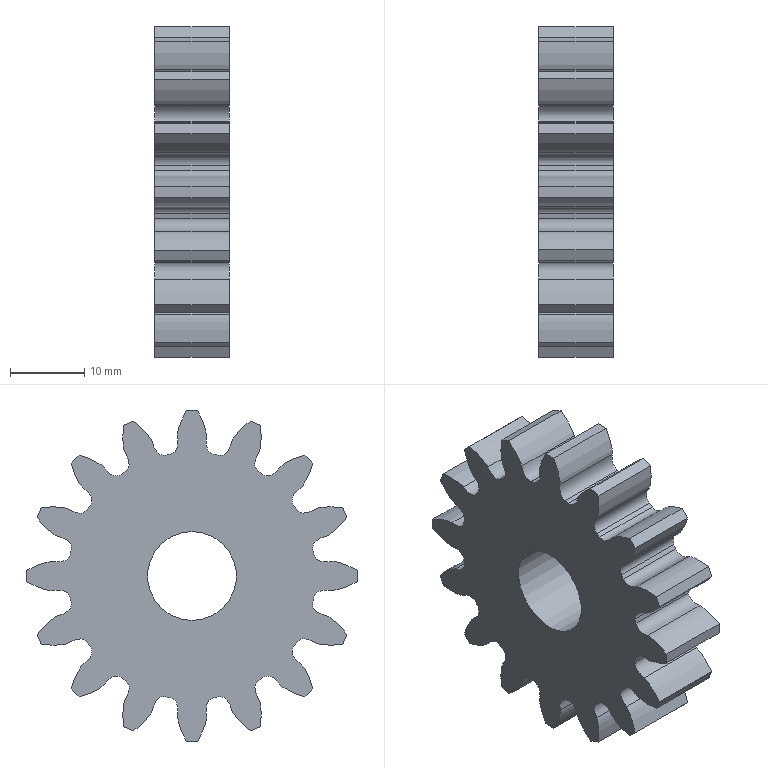Component | NX | IDLER_GEAR | 1 solid | 99 faces | volume 10783 mm3 | spline 80 | cylinder 17 | plane 2 | commonest cylinder face diameters 33.45 x16 12 x1